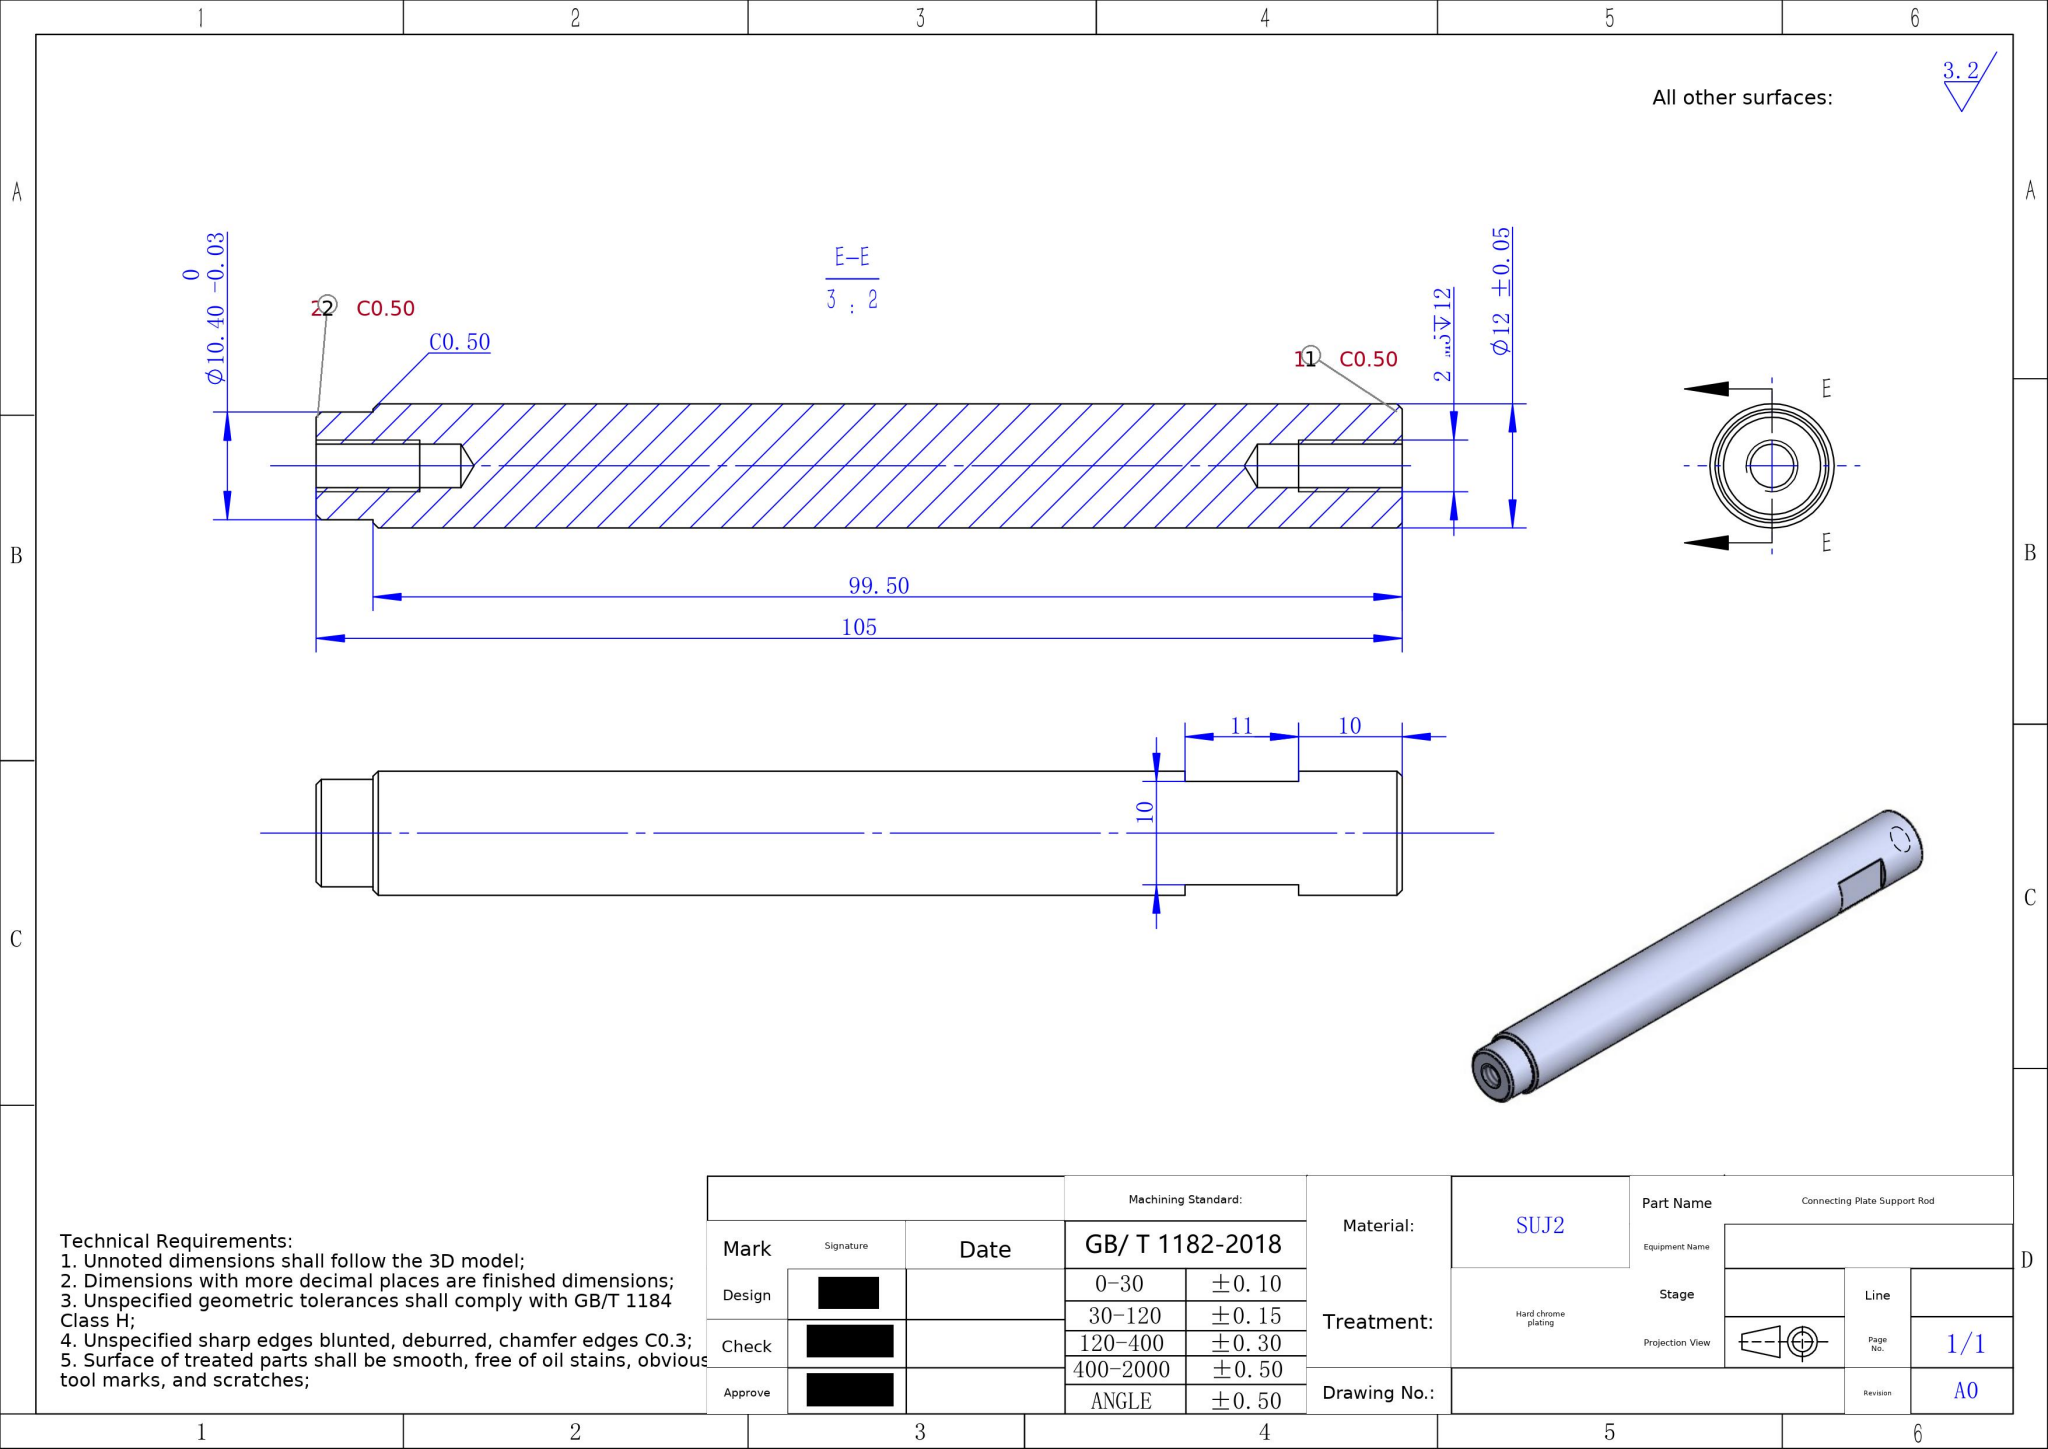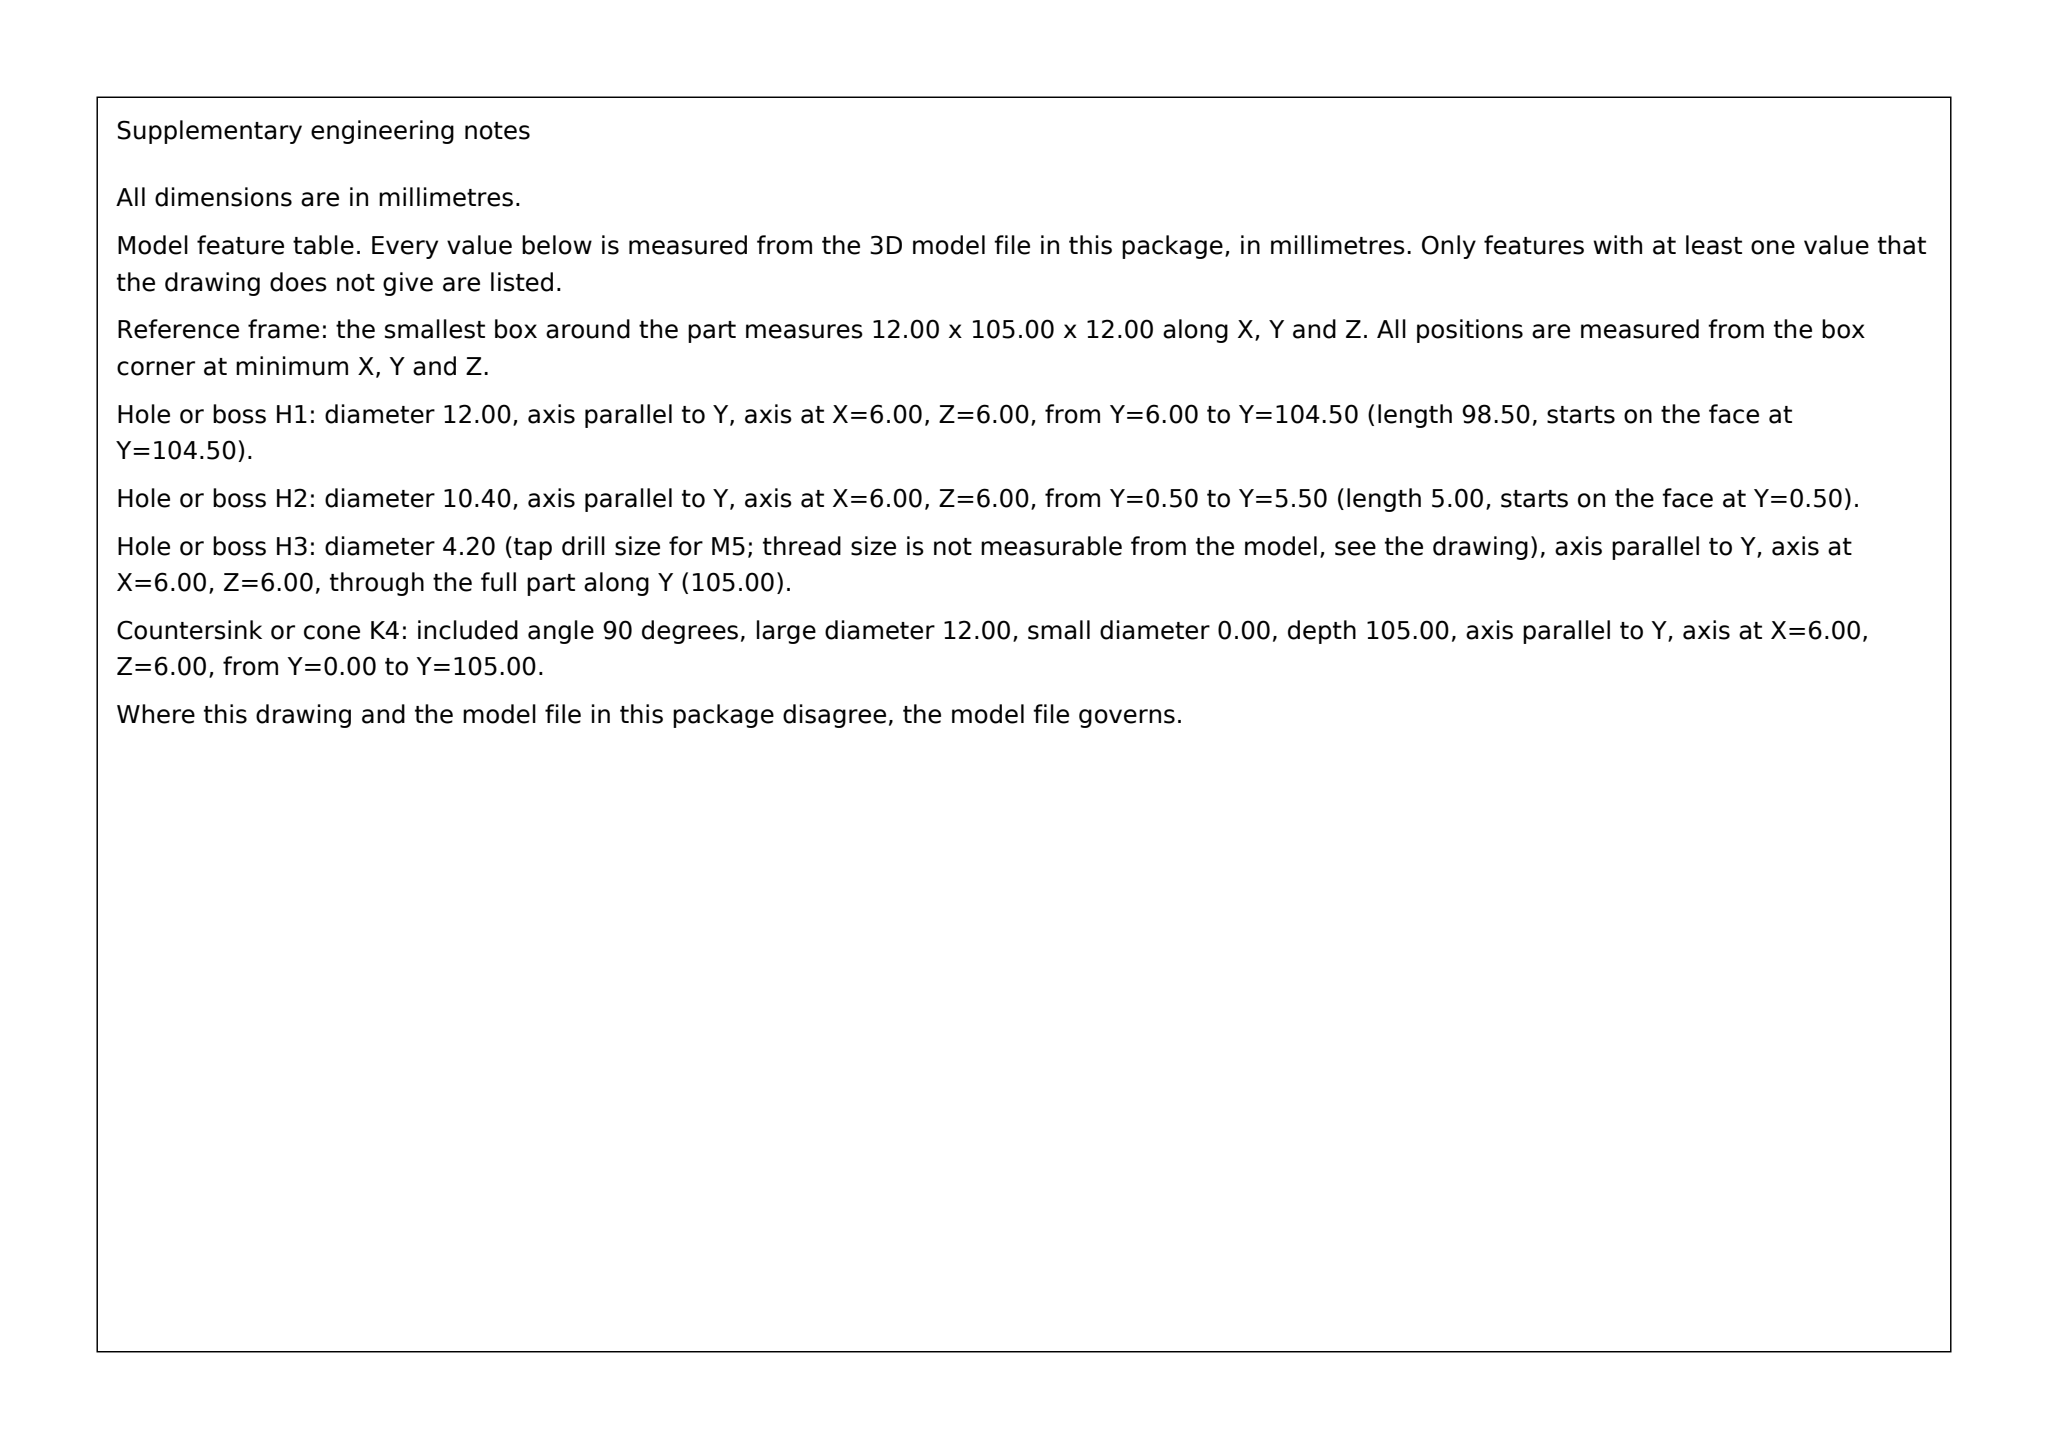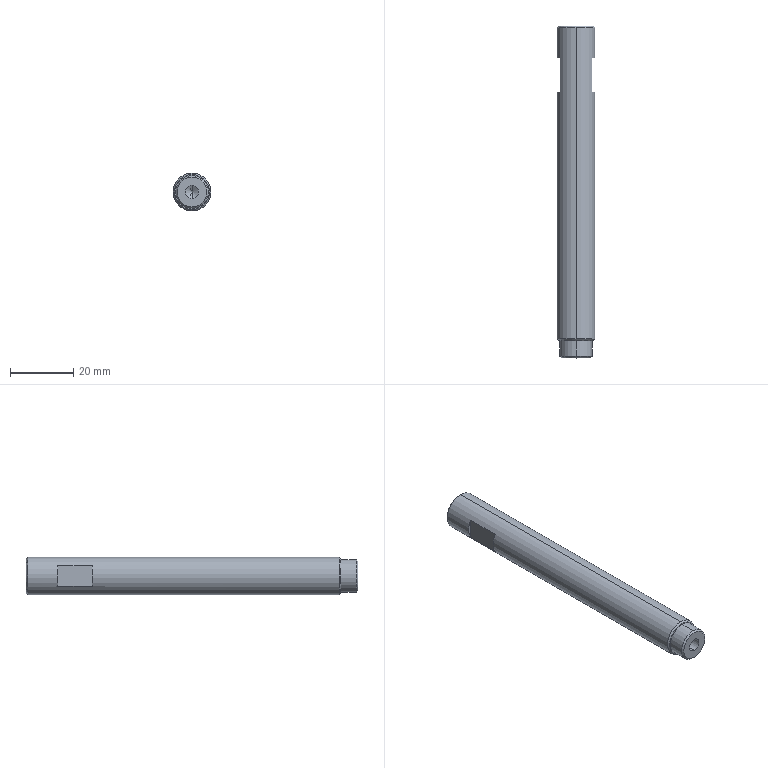Part | SolidWorks | mm | material SUJ2 | 1 solid | 27 faces | box 12 x 105 x 12 mm | volume 11209 mm3 | cone 10 | plane 9 | cylinder 8 | commonest cylinder face diameters 4.2 x4 10.4 x2 12 x2
build123d program:
from build123d import *

# Parameters (mm, degrees)
SKETCH2_W             = 7.253
SKETCH2_H             = 11
CUT_EXTRUDE1_DEPTH    = 15
CHAMFER1_SIZE         = 0.5
M5_TAPPED_HOLE1_D     = 4.2
M5_TAPPED_HOLE1_DEPTH = 14
M5_TAPPED_HOLE1_TIP   = 1.262
M5_TAPPED_HOLE2_D     = 4.2
M5_TAPPED_HOLE2_DEPTH = 14
M5_TAPPED_HOLE2_TIP   = 1.262


with BuildPart() as part:
    # Sketch1 → Revolve1 (revolve)
    with BuildSketch(Plane.XY, mode=Mode.PRIVATE) as revolve1_sk:
        Polygon((0, 0), (6, 0), (6, -10), (6, -21), (6, -99.5), (5.2, -99.5), (5.2, -105), (0, -105), align=None)
    revolve(revolve1_sk.sketch.rotate(Axis((0, 0, 0), (0, 1, 0)), 90), axis=Axis((0, 0, 0), (0, 1, 0)))

    # Sketch2 → Cut-Extrude1 (cut, symmetric)
    with BuildSketch(Plane.XY):
        with Locations((8.626, -15.5)):
            Rectangle(SKETCH2_W, SKETCH2_H)
        with Locations((-8.626, -15.5)):
            Rectangle(SKETCH2_W, SKETCH2_H)
    extrude(amount=CUT_EXTRUDE1_DEPTH, both=True, mode=Mode.SUBTRACT)

    # Chamfer1
    chamfer1_edges = [part.edges().sort_by_distance(p)[0] for p in [
        (0, -105, 5.2),
        (0, -99.5, 6),
        (0, 0, 6),
    ]]
    chamfer(chamfer1_edges, length=CHAMFER1_SIZE)

    # M5 Tapped Hole1
    with Locations(Plane(origin=(0, -105, 0), x_dir=(-1, 0, 0), z_dir=(0, -1, 0))):
        with Locations((0, 0)):
            Hole(M5_TAPPED_HOLE1_D / 2, depth=M5_TAPPED_HOLE1_DEPTH)
            with Locations((0, 0, -(M5_TAPPED_HOLE1_DEPTH + M5_TAPPED_HOLE1_TIP / 2))):  # 118° drill point
                Cone(0, M5_TAPPED_HOLE1_D / 2, M5_TAPPED_HOLE1_TIP, mode=Mode.SUBTRACT)

    # M5 Tapped Hole2
    with Locations(Plane(origin=(0, 0, 0), x_dir=(1, 0, 0), z_dir=(0, 1, 0))):
        with Locations((0, 0)):
            Hole(M5_TAPPED_HOLE2_D / 2, depth=M5_TAPPED_HOLE2_DEPTH)
            with Locations((0, 0, -(M5_TAPPED_HOLE2_DEPTH + M5_TAPPED_HOLE2_TIP / 2))):  # 118° drill point
                Cone(0, M5_TAPPED_HOLE2_D / 2, M5_TAPPED_HOLE2_TIP, mode=Mode.SUBTRACT)


solid = part.part
STEP:
#1=CARTESIAN_POINT('',(0.,-14.,-2.1));
#2=VERTEX_POINT('',#1);
#3=CARTESIAN_POINT('',(0.,-14.,2.1));
#4=VERTEX_POINT('',#3);
#5=CARTESIAN_POINT('',(0.,-14.,0.));
#6=DIRECTION('',(0.,1.,0.));
#7=DIRECTION('',(0.,0.,1.));
#8=AXIS2_PLACEMENT_3D('',#5,#6,#7);
#9=CIRCLE('',#8,2.1);
#10=EDGE_CURVE('',#2,#4,#9,.T.);
#11=ORIENTED_EDGE('',*,*,#10,.F.);
#12=CARTESIAN_POINT('',(0.,0.,-2.1));
#13=VERTEX_POINT('',#12);
#14=CARTESIAN_POINT('',(0.,0.,-2.1));
#15=DIRECTION('',(0.,1.,0.));
#16=VECTOR('',#15,1000.);
#17=LINE('',#14,#16);
#18=EDGE_CURVE('',#2,#13,#17,.T.);
#19=ORIENTED_EDGE('',*,*,#18,.T.);
#20=CARTESIAN_POINT('',(0.,0.,2.1));
#21=VERTEX_POINT('',#20);
#22=CARTESIAN_POINT('',(0.,0.,0.));
#23=DIRECTION('',(0.,1.,0.));
#24=DIRECTION('',(0.,0.,1.));
#25=AXIS2_PLACEMENT_3D('',#22,#23,#24);
#26=CIRCLE('',#25,2.1);
#27=EDGE_CURVE('',#13,#21,#26,.T.);
#28=ORIENTED_EDGE('',*,*,#27,.T.);
#29=CARTESIAN_POINT('',(0.,0.,2.1));
#30=DIRECTION('',(0.,1.,0.));
#31=VECTOR('',#30,1000.);
#32=LINE('',#29,#31);
#33=EDGE_CURVE('',#4,#21,#32,.T.);
#34=ORIENTED_EDGE('',*,*,#33,.F.);
#35=EDGE_LOOP('',(#11,#19,#28,#34));
#36=FACE_OUTER_BOUND('',#35,.T.);
#37=CARTESIAN_POINT('',(0.,0.,0.));
#38=DIRECTION('',(0.,1.,0.));
#39=DIRECTION('',(0.,0.,1.));
#40=AXIS2_PLACEMENT_3D('',#37,#38,#39);
#41=CYLINDRICAL_SURFACE('',#40,2.1);
#42=ADVANCED_FACE('',(#36),#41,.F.);
#43=CARTESIAN_POINT('',(-0.,-15.262,0.));
#44=VERTEX_POINT('',#43);
#45=CARTESIAN_POINT('',(0.,-14.,2.1));
#46=DIRECTION('',(0.,0.515,0.8572));
#47=VECTOR('',#46,1000.);
#48=LINE('',#45,#47);
#49=EDGE_CURVE('',#44,#4,#48,.T.);
#50=ORIENTED_EDGE('',*,*,#49,.F.);
#51=CARTESIAN_POINT('',(0.,-14.,-2.1));
#52=DIRECTION('',(0.,0.515,-0.8572));
#53=VECTOR('',#52,1000.);
#54=LINE('',#51,#53);
#55=EDGE_CURVE('',#44,#2,#54,.T.);
#56=ORIENTED_EDGE('',*,*,#55,.T.);
#57=ORIENTED_EDGE('',*,*,#10,.T.);
#58=EDGE_LOOP('',(#50,#56,#57));
#59=FACE_OUTER_BOUND('',#58,.T.);
#60=CARTESIAN_POINT('',(0.,-14.,0.));
#61=DIRECTION('',(0.,1.,0.));
#62=DIRECTION('',(0.,0.,1.));
#63=AXIS2_PLACEMENT_3D('',#60,#61,#62);
#64=CONICAL_SURFACE('',#63,2.1,1.03);
#65=ADVANCED_FACE('',(#59),#64,.F.);
#66=CARTESIAN_POINT('',(0.,-91.,2.1));
#67=VERTEX_POINT('',#66);
#68=CARTESIAN_POINT('',(0.,-91.,-2.1));
#69=VERTEX_POINT('',#68);
#70=CARTESIAN_POINT('',(0.,-91.,0.));
#71=DIRECTION('',(0.,-1.,0.));
#72=DIRECTION('',(0.,0.,-1.));
#73=AXIS2_PLACEMENT_3D('',#70,#71,#72);
#74=CIRCLE('',#73,2.1);
#75=EDGE_CURVE('',#67,#69,#74,.T.);
#76=ORIENTED_EDGE('',*,*,#75,.F.);
#77=CARTESIAN_POINT('',(0.,-105.,2.1));
#78=VERTEX_POINT('',#77);
#79=CARTESIAN_POINT('',(0.,-105.,2.1));
#80=DIRECTION('',(0.,-1.,0.));
#81=VECTOR('',#80,1000.);
#82=LINE('',#79,#81);
#83=EDGE_CURVE('',#67,#78,#82,.T.);
#84=ORIENTED_EDGE('',*,*,#83,.T.);
#85=CARTESIAN_POINT('',(0.,-105.,-2.1));
#86=VERTEX_POINT('',#85);
#87=CARTESIAN_POINT('',(0.,-105.,0.));
#88=DIRECTION('',(0.,-1.,0.));
#89=DIRECTION('',(0.,0.,-1.));
#90=AXIS2_PLACEMENT_3D('',#87,#88,#89);
#91=CIRCLE('',#90,2.1);
#92=EDGE_CURVE('',#78,#86,#91,.T.);
#93=ORIENTED_EDGE('',*,*,#92,.T.);
#94=CARTESIAN_POINT('',(0.,-105.,-2.1));
#95=DIRECTION('',(0.,-1.,0.));
#96=VECTOR('',#95,1000.);
#97=LINE('',#94,#96);
#98=EDGE_CURVE('',#69,#86,#97,.T.);
#99=ORIENTED_EDGE('',*,*,#98,.F.);
#100=EDGE_LOOP('',(#76,#84,#93,#99));
#101=FACE_OUTER_BOUND('',#100,.T.);
#102=CARTESIAN_POINT('',(0.,-105.,0.));
#103=DIRECTION('',(0.,-1.,0.));
#104=DIRECTION('',(0.,0.,-1.));
#105=AXIS2_PLACEMENT_3D('',#102,#103,#104);
#106=CYLINDRICAL_SURFACE('',#105,2.1);
#107=ADVANCED_FACE('',(#101),#106,.F.);
#108=CARTESIAN_POINT('',(-0.,-89.738,0.));
#109=VERTEX_POINT('',#108);
#110=CARTESIAN_POINT('',(0.,-91.,-2.1));
#111=DIRECTION('',(0.,-0.515,-0.8572));
#112=VECTOR('',#111,1000.);
#113=LINE('',#110,#112);
#114=EDGE_CURVE('',#109,#69,#113,.T.);
#115=ORIENTED_EDGE('',*,*,#114,.F.);
#116=CARTESIAN_POINT('',(0.,-91.,2.1));
#117=DIRECTION('',(0.,-0.515,0.8572));
#118=VECTOR('',#117,1000.);
#119=LINE('',#116,#118);
#120=EDGE_CURVE('',#109,#67,#119,.T.);
#121=ORIENTED_EDGE('',*,*,#120,.T.);
#122=ORIENTED_EDGE('',*,*,#75,.T.);
#123=EDGE_LOOP('',(#115,#121,#122));
#124=FACE_OUTER_BOUND('',#123,.T.);
#125=CARTESIAN_POINT('',(0.,-91.,0.));
#126=DIRECTION('',(0.,-1.,0.));
#127=DIRECTION('',(0.,0.,-1.));
#128=AXIS2_PLACEMENT_3D('',#125,#126,#127);
#129=CONICAL_SURFACE('',#128,2.1,1.03);
#130=ADVANCED_FACE('',(#124),#129,.F.);
#131=CARTESIAN_POINT('',(0.,-0.,5.5));
#132=VERTEX_POINT('',#131);
#133=CARTESIAN_POINT('',(0.,-0.,-5.5));
#134=VERTEX_POINT('',#133);
#135=CARTESIAN_POINT('',(0.,-0.,0.));
#136=DIRECTION('',(0.,1.,0.));
#137=DIRECTION('',(0.,0.,1.));
#138=AXIS2_PLACEMENT_3D('',#135,#136,#137);
#139=CIRCLE('',#138,5.5);
#140=EDGE_CURVE('',#132,#134,#139,.T.);
#141=ORIENTED_EDGE('',*,*,#140,.F.);
#142=CARTESIAN_POINT('',(0.,-0.5,6.));
#143=VERTEX_POINT('',#142);
#144=CARTESIAN_POINT('',(0.,-0.5,6.));
#145=DIRECTION('',(0.,-0.7071,0.7071));
#146=VECTOR('',#145,1000.);
#147=LINE('',#144,#146);
#148=EDGE_CURVE('',#132,#143,#147,.T.);
#149=ORIENTED_EDGE('',*,*,#148,.T.);
#150=CARTESIAN_POINT('',(0.,-0.5,-6.));
#151=VERTEX_POINT('',#150);
#152=CARTESIAN_POINT('',(0.,-0.5,0.));
#153=DIRECTION('',(0.,-1.,0.));
#154=DIRECTION('',(0.,0.,1.));
#155=AXIS2_PLACEMENT_3D('',#152,#153,#154);
#156=CIRCLE('',#155,6.);
#157=EDGE_CURVE('',#151,#143,#156,.T.);
#158=ORIENTED_EDGE('',*,*,#157,.F.);
#159=CARTESIAN_POINT('',(0.,-0.5,-6.));
#160=DIRECTION('',(0.,-0.7071,-0.7071));
#161=VECTOR('',#160,1000.);
#162=LINE('',#159,#161);
#163=EDGE_CURVE('',#134,#151,#162,.T.);
#164=ORIENTED_EDGE('',*,*,#163,.F.);
#165=EDGE_LOOP('',(#141,#149,#158,#164));
#166=FACE_OUTER_BOUND('',#165,.T.);
#167=CARTESIAN_POINT('',(0.,-0.5,0.));
#168=DIRECTION('',(0.,-1.,0.));
#169=DIRECTION('',(0.,0.,-1.));
#170=AXIS2_PLACEMENT_3D('',#167,#168,#169);
#171=CONICAL_SURFACE('',#170,6.,0.7854);
#172=ADVANCED_FACE('',(#166),#171,.T.);
#173=CARTESIAN_POINT('',(0.,-99.5,-5.5));
#174=VERTEX_POINT('',#173);
#175=CARTESIAN_POINT('',(0.,-99.5,5.5));
#176=VERTEX_POINT('',#175);
#177=CARTESIAN_POINT('',(0.,-99.5,0.));
#178=DIRECTION('',(0.,-1.,0.));
#179=DIRECTION('',(0.,0.,-1.));
#180=AXIS2_PLACEMENT_3D('',#177,#178,#179);
#181=CIRCLE('',#180,5.5);
#182=EDGE_CURVE('',#174,#176,#181,.T.);
#183=ORIENTED_EDGE('',*,*,#182,.F.);
#184=CARTESIAN_POINT('',(0.,-99.,-6.));
#185=VERTEX_POINT('',#184);
#186=CARTESIAN_POINT('',(0.,-99.5,-5.5));
#187=DIRECTION('',(0.,0.7071,-0.7071));
#188=VECTOR('',#187,1000.);
#189=LINE('',#186,#188);
#190=EDGE_CURVE('',#174,#185,#189,.T.);
#191=ORIENTED_EDGE('',*,*,#190,.T.);
#192=CARTESIAN_POINT('',(0.,-99.,6.));
#193=VERTEX_POINT('',#192);
#194=CARTESIAN_POINT('',(0.,-99.,0.));
#195=DIRECTION('',(0.,1.,0.));
#196=DIRECTION('',(0.,0.,-1.));
#197=AXIS2_PLACEMENT_3D('',#194,#195,#196);
#198=CIRCLE('',#197,6.);
#199=EDGE_CURVE('',#193,#185,#198,.T.);
#200=ORIENTED_EDGE('',*,*,#199,.F.);
#201=CARTESIAN_POINT('',(0.,-99.5,5.5));
#202=DIRECTION('',(0.,0.7071,0.7071));
#203=VECTOR('',#202,1000.);
#204=LINE('',#201,#203);
#205=EDGE_CURVE('',#176,#193,#204,.T.);
#206=ORIENTED_EDGE('',*,*,#205,.F.);
#207=EDGE_LOOP('',(#183,#191,#200,#206));
#208=FACE_OUTER_BOUND('',#207,.T.);
#209=CARTESIAN_POINT('',(0.,-99.5,0.));
#210=DIRECTION('',(0.,1.,0.));
#211=DIRECTION('',(0.,0.,1.));
#212=AXIS2_PLACEMENT_3D('',#209,#210,#211);
#213=CONICAL_SURFACE('',#212,5.5,0.7854);
#214=ADVANCED_FACE('',(#208),#213,.T.);
#215=CARTESIAN_POINT('',(0.,-105.,-4.7));
#216=VERTEX_POINT('',#215);
#217=CARTESIAN_POINT('',(0.,-105.,4.7));
#218=VERTEX_POINT('',#217);
#219=CARTESIAN_POINT('',(0.,-105.,0.));
#220=DIRECTION('',(0.,-1.,0.));
#221=DIRECTION('',(0.,0.,-1.));
#222=AXIS2_PLACEMENT_3D('',#219,#220,#221);
#223=CIRCLE('',#222,4.7);
#224=EDGE_CURVE('',#216,#218,#223,.T.);
#225=ORIENTED_EDGE('',*,*,#224,.F.);
#226=CARTESIAN_POINT('',(0.,-104.5,-5.2));
#227=VERTEX_POINT('',#226);
#228=CARTESIAN_POINT('',(0.,-105.,-4.7));
#229=DIRECTION('',(0.,0.7071,-0.7071));
#230=VECTOR('',#229,1000.);
#231=LINE('',#228,#230);
#232=EDGE_CURVE('',#216,#227,#231,.T.);
#233=ORIENTED_EDGE('',*,*,#232,.T.);
#234=CARTESIAN_POINT('',(0.,-104.5,5.2));
#235=VERTEX_POINT('',#234);
#236=CARTESIAN_POINT('',(0.,-104.5,0.));
#237=DIRECTION('',(0.,1.,0.));
#238=DIRECTION('',(0.,0.,-1.));
#239=AXIS2_PLACEMENT_3D('',#236,#237,#238);
#240=CIRCLE('',#239,5.2);
#241=EDGE_CURVE('',#235,#227,#240,.T.);
#242=ORIENTED_EDGE('',*,*,#241,.F.);
#243=CARTESIAN_POINT('',(0.,-105.,4.7));
#244=DIRECTION('',(0.,0.7071,0.7071));
#245=VECTOR('',#244,1000.);
#246=LINE('',#243,#245);
#247=EDGE_CURVE('',#218,#235,#246,.T.);
#248=ORIENTED_EDGE('',*,*,#247,.F.);
#249=EDGE_LOOP('',(#225,#233,#242,#248));
#250=FACE_OUTER_BOUND('',#249,.T.);
#251=CARTESIAN_POINT('',(0.,-105.,0.));
#252=DIRECTION('',(0.,1.,0.));
#253=DIRECTION('',(0.,0.,1.));
#254=AXIS2_PLACEMENT_3D('',#251,#252,#253);
#255=CONICAL_SURFACE('',#254,4.7,0.7854);
#256=ADVANCED_FACE('',(#250),#255,.T.);
#257=CARTESIAN_POINT('',(0.,-99.5,-5.2));
#258=VERTEX_POINT('',#257);
#259=CARTESIAN_POINT('',(0.,-99.5,5.2));
#260=VERTEX_POINT('',#259);
#261=CARTESIAN_POINT('',(0.,-99.5,0.));
#262=DIRECTION('',(0.,-1.,0.));
#263=DIRECTION('',(0.,0.,-1.));
#264=AXIS2_PLACEMENT_3D('',#261,#262,#263);
#265=CIRCLE('',#264,5.2);
#266=EDGE_CURVE('',#258,#260,#265,.T.);
#267=ORIENTED_EDGE('',*,*,#266,.T.);
#268=CARTESIAN_POINT('',(0.,0.,5.2));
#269=DIRECTION('',(0.,-1.,0.));
#270=VECTOR('',#269,1000.);
#271=LINE('',#268,#270);
#272=EDGE_CURVE('',#260,#235,#271,.T.);
#273=ORIENTED_EDGE('',*,*,#272,.T.);
#274=ORIENTED_EDGE('',*,*,#241,.T.);
#275=CARTESIAN_POINT('',(0.,0.,-5.2));
#276=DIRECTION('',(0.,-1.,0.));
#277=VECTOR('',#276,1000.);
#278=LINE('',#275,#277);
#279=EDGE_CURVE('',#258,#227,#278,.T.);
#280=ORIENTED_EDGE('',*,*,#279,.F.);
#281=EDGE_LOOP('',(#267,#273,#274,#280));
#282=FACE_OUTER_BOUND('',#281,.T.);
#283=CARTESIAN_POINT('',(0.,0.,0.));
#284=DIRECTION('',(0.,-1.,0.));
#285=DIRECTION('',(0.,0.,-1.));
#286=AXIS2_PLACEMENT_3D('',#283,#284,#285);
#287=CYLINDRICAL_SURFACE('',#286,5.2);
#288=ADVANCED_FACE('',(#282),#287,.T.);
#289=CARTESIAN_POINT('',(5.,-21.,3.317));
#290=VERTEX_POINT('',#289);
#291=CARTESIAN_POINT('',(5.,-21.,-3.317));
#292=VERTEX_POINT('',#291);
#293=CARTESIAN_POINT('',(0.,-21.,0.));
#294=DIRECTION('',(0.,1.,0.));
#295=DIRECTION('',(-0.,0.,-1.));
#296=AXIS2_PLACEMENT_3D('',#293,#294,#295);
#297=CIRCLE('',#296,6.);
#298=EDGE_CURVE('',#290,#292,#297,.T.);
#299=ORIENTED_EDGE('',*,*,#298,.F.);
#300=CARTESIAN_POINT('',(5.,-10.,3.317));
#301=VERTEX_POINT('',#300);
#302=CARTESIAN_POINT('',(5.,0.,3.317));
#303=DIRECTION('',(0.,-1.,0.));
#304=VECTOR('',#303,1000.);
#305=LINE('',#302,#304);
#306=EDGE_CURVE('',#301,#290,#305,.T.);
#307=ORIENTED_EDGE('',*,*,#306,.F.);
#308=CARTESIAN_POINT('',(5.,-10.,-3.317));
#309=VERTEX_POINT('',#308);
#310=CARTESIAN_POINT('',(0.,-10.,0.));
#311=DIRECTION('',(-0.,-1.,0.));
#312=DIRECTION('',(-1.,0.,0.));
#313=AXIS2_PLACEMENT_3D('',#310,#311,#312);
#314=CIRCLE('',#313,6.);
#315=EDGE_CURVE('',#309,#301,#314,.T.);
#316=ORIENTED_EDGE('',*,*,#315,.F.);
#317=CARTESIAN_POINT('',(5.,0.,-3.317));
#318=DIRECTION('',(0.,1.,0.));
#319=VECTOR('',#318,1000.);
#320=LINE('',#317,#319);
#321=EDGE_CURVE('',#292,#309,#320,.T.);
#322=ORIENTED_EDGE('',*,*,#321,.F.);
#323=EDGE_LOOP('',(#299,#307,#316,#322));
#324=FACE_BOUND('',#323,.T.);
#325=ORIENTED_EDGE('',*,*,#157,.T.);
#326=CARTESIAN_POINT('',(0.,0.,6.));
#327=DIRECTION('',(0.,-1.,0.));
#328=VECTOR('',#327,1000.);
#329=LINE('',#326,#328);
#330=EDGE_CURVE('',#143,#193,#329,.T.);
#331=ORIENTED_EDGE('',*,*,#330,.T.);
#332=ORIENTED_EDGE('',*,*,#199,.T.);
#333=CARTESIAN_POINT('',(0.,0.,-6.));
#334=DIRECTION('',(0.,-1.,0.));
#335=VECTOR('',#334,1000.);
#336=LINE('',#333,#335);
#337=EDGE_CURVE('',#151,#185,#336,.T.);
#338=ORIENTED_EDGE('',*,*,#337,.F.);
#339=EDGE_LOOP('',(#325,#331,#332,#338));
#340=FACE_OUTER_BOUND('',#339,.T.);
#341=CARTESIAN_POINT('',(0.,0.,0.));
#342=DIRECTION('',(0.,-1.,0.));
#343=DIRECTION('',(0.,0.,-1.));
#344=AXIS2_PLACEMENT_3D('',#341,#342,#343);
#345=CYLINDRICAL_SURFACE('',#344,6.);
#346=ADVANCED_FACE('',(#324,#340),#345,.T.);
#347=CARTESIAN_POINT('',(0.,0.,0.));
#348=DIRECTION('',(0.,1.,0.));
#349=DIRECTION('',(0.,0.,1.));
#350=AXIS2_PLACEMENT_3D('',#347,#348,#349);
#351=CIRCLE('',#350,2.1);
#352=EDGE_CURVE('',#21,#13,#351,.T.);
#353=ORIENTED_EDGE('',*,*,#352,.F.);
#354=ORIENTED_EDGE('',*,*,#27,.F.);
#355=EDGE_LOOP('',(#353,#354));
#356=FACE_BOUND('',#355,.T.);
#357=CARTESIAN_POINT('',(0.,-0.,0.));
#358=DIRECTION('',(0.,1.,0.));
#359=DIRECTION('',(0.,0.,1.));
#360=AXIS2_PLACEMENT_3D('',#357,#358,#359);
#361=CIRCLE('',#360,5.5);
#362=EDGE_CURVE('',#134,#132,#361,.T.);
#363=ORIENTED_EDGE('',*,*,#362,.T.);
#364=ORIENTED_EDGE('',*,*,#140,.T.);
#365=EDGE_LOOP('',(#363,#364));
#366=FACE_OUTER_BOUND('',#365,.T.);
#367=CARTESIAN_POINT('',(0.,-0.,0.));
#368=DIRECTION('',(0.,1.,0.));
#369=DIRECTION('',(0.,0.,1.));
#370=AXIS2_PLACEMENT_3D('',#367,#368,#369);
#371=PLANE('',#370);
#372=ADVANCED_FACE('',(#356,#366),#371,.T.);
#373=ORIENTED_EDGE('',*,*,#330,.F.);
#374=CARTESIAN_POINT('',(0.,-0.5,0.));
#375=DIRECTION('',(0.,-1.,0.));
#376=DIRECTION('',(0.,0.,1.));
#377=AXIS2_PLACEMENT_3D('',#374,#375,#376);
#378=CIRCLE('',#377,6.);
#379=EDGE_CURVE('',#143,#151,#378,.T.);
#380=ORIENTED_EDGE('',*,*,#379,.T.);
#381=ORIENTED_EDGE('',*,*,#337,.T.);
#382=CARTESIAN_POINT('',(0.,-99.,0.));
#383=DIRECTION('',(0.,1.,0.));
#384=DIRECTION('',(0.,0.,-1.));
#385=AXIS2_PLACEMENT_3D('',#382,#383,#384);
#386=CIRCLE('',#385,6.);
#387=EDGE_CURVE('',#185,#193,#386,.T.);
#388=ORIENTED_EDGE('',*,*,#387,.T.);
#389=EDGE_LOOP('',(#373,#380,#381,#388));
#390=FACE_OUTER_BOUND('',#389,.T.);
#391=CARTESIAN_POINT('',(-5.,-10.,3.317));
#392=VERTEX_POINT('',#391);
#393=CARTESIAN_POINT('',(-5.,-10.,-3.317));
#394=VERTEX_POINT('',#393);
#395=CARTESIAN_POINT('',(0.,-10.,0.));
#396=DIRECTION('',(0.,-1.,0.));
#397=DIRECTION('',(-1.,-0.,0.));
#398=AXIS2_PLACEMENT_3D('',#395,#396,#397);
#399=CIRCLE('',#398,6.);
#400=EDGE_CURVE('',#392,#394,#399,.T.);
#401=ORIENTED_EDGE('',*,*,#400,.F.);
#402=CARTESIAN_POINT('',(-5.,-21.,3.317));
#403=VERTEX_POINT('',#402);
#404=CARTESIAN_POINT('',(-5.,0.,3.317));
#405=DIRECTION('',(0.,1.,0.));
#406=VECTOR('',#405,1000.);
#407=LINE('',#404,#406);
#408=EDGE_CURVE('',#403,#392,#407,.T.);
#409=ORIENTED_EDGE('',*,*,#408,.F.);
#410=CARTESIAN_POINT('',(-5.,-21.,-3.317));
#411=VERTEX_POINT('',#410);
#412=CARTESIAN_POINT('',(0.,-21.,0.));
#413=DIRECTION('',(0.,1.,0.));
#414=DIRECTION('',(0.,0.,-1.));
#415=AXIS2_PLACEMENT_3D('',#412,#413,#414);
#416=CIRCLE('',#415,6.);
#417=EDGE_CURVE('',#411,#403,#416,.T.);
#418=ORIENTED_EDGE('',*,*,#417,.F.);
#419=CARTESIAN_POINT('',(-5.,0.,-3.317));
#420=DIRECTION('',(0.,-1.,0.));
#421=VECTOR('',#420,1000.);
#422=LINE('',#419,#421);
#423=EDGE_CURVE('',#394,#411,#422,.T.);
#424=ORIENTED_EDGE('',*,*,#423,.F.);
#425=EDGE_LOOP('',(#401,#409,#418,#424));
#426=FACE_BOUND('',#425,.T.);
#427=CARTESIAN_POINT('',(0.,0.,0.));
#428=DIRECTION('',(0.,-1.,0.));
#429=DIRECTION('',(0.,0.,-1.));
#430=AXIS2_PLACEMENT_3D('',#427,#428,#429);
#431=CYLINDRICAL_SURFACE('',#430,6.);
#432=ADVANCED_FACE('',(#390,#426),#431,.T.);
#433=CARTESIAN_POINT('',(0.,-99.5,0.));
#434=DIRECTION('',(0.,-1.,0.));
#435=DIRECTION('',(0.,0.,-1.));
#436=AXIS2_PLACEMENT_3D('',#433,#434,#435);
#437=CIRCLE('',#436,5.5);
#438=EDGE_CURVE('',#176,#174,#437,.T.);
#439=ORIENTED_EDGE('',*,*,#438,.T.);
#440=ORIENTED_EDGE('',*,*,#182,.T.);
#441=EDGE_LOOP('',(#439,#440));
#442=FACE_OUTER_BOUND('',#441,.T.);
#443=ORIENTED_EDGE('',*,*,#266,.F.);
#444=CARTESIAN_POINT('',(0.,-99.5,0.));
#445=DIRECTION('',(0.,-1.,0.));
#446=DIRECTION('',(0.,0.,-1.));
#447=AXIS2_PLACEMENT_3D('',#444,#445,#446);
#448=CIRCLE('',#447,5.2);
#449=EDGE_CURVE('',#260,#258,#448,.T.);
#450=ORIENTED_EDGE('',*,*,#449,.F.);
#451=EDGE_LOOP('',(#443,#450));
#452=FACE_BOUND('',#451,.T.);
#453=CARTESIAN_POINT('',(6.,-99.5,0.));
#454=DIRECTION('',(0.,-1.,0.));
#455=DIRECTION('',(0.,0.,-1.));
#456=AXIS2_PLACEMENT_3D('',#453,#454,#455);
#457=PLANE('',#456);
#458=ADVANCED_FACE('',(#442,#452),#457,.T.);
#459=ORIENTED_EDGE('',*,*,#272,.F.);
#460=ORIENTED_EDGE('',*,*,#449,.T.);
#461=ORIENTED_EDGE('',*,*,#279,.T.);
#462=CARTESIAN_POINT('',(0.,-104.5,0.));
#463=DIRECTION('',(0.,1.,0.));
#464=DIRECTION('',(0.,0.,-1.));
#465=AXIS2_PLACEMENT_3D('',#462,#463,#464);
#466=CIRCLE('',#465,5.2);
#467=EDGE_CURVE('',#227,#235,#466,.T.);
#468=ORIENTED_EDGE('',*,*,#467,.T.);
#469=EDGE_LOOP('',(#459,#460,#461,#468));
#470=FACE_OUTER_BOUND('',#469,.T.);
#471=CARTESIAN_POINT('',(0.,0.,0.));
#472=DIRECTION('',(0.,-1.,0.));
#473=DIRECTION('',(0.,0.,-1.));
#474=AXIS2_PLACEMENT_3D('',#471,#472,#473);
#475=CYLINDRICAL_SURFACE('',#474,5.2);
#476=ADVANCED_FACE('',(#470),#475,.T.);
#477=CARTESIAN_POINT('',(0.,-105.,0.));
#478=DIRECTION('',(0.,-1.,0.));
#479=DIRECTION('',(0.,0.,-1.));
#480=AXIS2_PLACEMENT_3D('',#477,#478,#479);
#481=CIRCLE('',#480,2.1);
#482=EDGE_CURVE('',#86,#78,#481,.T.);
#483=ORIENTED_EDGE('',*,*,#482,.F.);
#484=ORIENTED_EDGE('',*,*,#92,.F.);
#485=EDGE_LOOP('',(#483,#484));
#486=FACE_BOUND('',#485,.T.);
#487=CARTESIAN_POINT('',(0.,-105.,0.));
#488=DIRECTION('',(0.,-1.,0.));
#489=DIRECTION('',(0.,0.,-1.));
#490=AXIS2_PLACEMENT_3D('',#487,#488,#489);
#491=CIRCLE('',#490,4.7);
#492=EDGE_CURVE('',#218,#216,#491,.T.);
#493=ORIENTED_EDGE('',*,*,#492,.T.);
#494=ORIENTED_EDGE('',*,*,#224,.T.);
#495=EDGE_LOOP('',(#493,#494));
#496=FACE_OUTER_BOUND('',#495,.T.);
#497=CARTESIAN_POINT('',(5.2,-105.,0.));
#498=DIRECTION('',(0.,-1.,0.));
#499=DIRECTION('',(0.,0.,-1.));
#500=AXIS2_PLACEMENT_3D('',#497,#498,#499);
#501=PLANE('',#500);
#502=ADVANCED_FACE('',(#486,#496),#501,.T.);
#503=ORIENTED_EDGE('',*,*,#400,.T.);
#504=CARTESIAN_POINT('',(-5.,-10.,-15.));
#505=DIRECTION('',(0.,0.,1.));
#506=VECTOR('',#505,1000.);
#507=LINE('',#504,#506);
#508=EDGE_CURVE('',#394,#392,#507,.T.);
#509=ORIENTED_EDGE('',*,*,#508,.T.);
#510=EDGE_LOOP('',(#503,#509));
#511=FACE_OUTER_BOUND('',#510,.T.);
#512=CARTESIAN_POINT('',(-12.253,-10.,-15.));
#513=DIRECTION('',(-0.,1.,0.));
#514=DIRECTION('',(-1.,-0.,0.));
#515=AXIS2_PLACEMENT_3D('',#512,#513,#514);
#516=PLANE('',#515);
#517=ADVANCED_FACE('',(#511),#516,.F.);
#518=ORIENTED_EDGE('',*,*,#408,.T.);
#519=ORIENTED_EDGE('',*,*,#508,.F.);
#520=ORIENTED_EDGE('',*,*,#423,.T.);
#521=CARTESIAN_POINT('',(-5.,-21.,-15.));
#522=DIRECTION('',(0.,0.,1.));
#523=VECTOR('',#522,1000.);
#524=LINE('',#521,#523);
#525=EDGE_CURVE('',#411,#403,#524,.T.);
#526=ORIENTED_EDGE('',*,*,#525,.T.);
#527=EDGE_LOOP('',(#518,#519,#520,#526));
#528=FACE_OUTER_BOUND('',#527,.T.);
#529=CARTESIAN_POINT('',(-5.,-10.,-15.));
#530=DIRECTION('',(1.,-0.,0.));
#531=DIRECTION('',(0.,1.,0.));
#532=AXIS2_PLACEMENT_3D('',#529,#530,#531);
#533=PLANE('',#532);
#534=ADVANCED_FACE('',(#528),#533,.F.);
#535=ORIENTED_EDGE('',*,*,#417,.T.);
#536=ORIENTED_EDGE('',*,*,#525,.F.);
#537=EDGE_LOOP('',(#535,#536));
#538=FACE_OUTER_BOUND('',#537,.T.);
#539=CARTESIAN_POINT('',(-12.253,-21.,-15.));
#540=DIRECTION('',(0.,-1.,0.));
#541=DIRECTION('',(0.,0.,-1.));
#542=AXIS2_PLACEMENT_3D('',#539,#540,#541);
#543=PLANE('',#542);
#544=ADVANCED_FACE('',(#538),#543,.F.);
#545=ORIENTED_EDGE('',*,*,#298,.T.);
#546=CARTESIAN_POINT('',(5.,-21.,-15.));
#547=DIRECTION('',(0.,0.,1.));
#548=VECTOR('',#547,1000.);
#549=LINE('',#546,#548);
#550=EDGE_CURVE('',#292,#290,#549,.T.);
#551=ORIENTED_EDGE('',*,*,#550,.T.);
#552=EDGE_LOOP('',(#545,#551));
#553=FACE_OUTER_BOUND('',#552,.T.);
#554=CARTESIAN_POINT('',(12.253,-21.,-15.));
#555=DIRECTION('',(0.,-1.,0.));
#556=DIRECTION('',(0.,0.,-1.));
#557=AXIS2_PLACEMENT_3D('',#554,#555,#556);
#558=PLANE('',#557);
#559=ADVANCED_FACE('',(#553),#558,.F.);
#560=ORIENTED_EDGE('',*,*,#321,.T.);
#561=CARTESIAN_POINT('',(5.,-10.,-15.));
#562=DIRECTION('',(0.,0.,1.));
#563=VECTOR('',#562,1000.);
#564=LINE('',#561,#563);
#565=EDGE_CURVE('',#309,#301,#564,.T.);
#566=ORIENTED_EDGE('',*,*,#565,.T.);
#567=ORIENTED_EDGE('',*,*,#306,.T.);
#568=ORIENTED_EDGE('',*,*,#550,.F.);
#569=EDGE_LOOP('',(#560,#566,#567,#568));
#570=FACE_OUTER_BOUND('',#569,.T.);
#571=CARTESIAN_POINT('',(5.,-10.,-15.));
#572=DIRECTION('',(-1.,-0.,0.));
#573=DIRECTION('',(0.,-1.,0.));
#574=AXIS2_PLACEMENT_3D('',#571,#572,#573);
#575=PLANE('',#574);
#576=ADVANCED_FACE('',(#570),#575,.F.);
#577=ORIENTED_EDGE('',*,*,#315,.T.);
#578=ORIENTED_EDGE('',*,*,#565,.F.);
#579=EDGE_LOOP('',(#577,#578));
#580=FACE_OUTER_BOUND('',#579,.T.);
#581=CARTESIAN_POINT('',(12.253,-10.,-15.));
#582=DIRECTION('',(0.,1.,0.));
#583=DIRECTION('',(-1.,0.,0.));
#584=AXIS2_PLACEMENT_3D('',#581,#582,#583);
#585=PLANE('',#584);
#586=ADVANCED_FACE('',(#580),#585,.F.);
#587=ORIENTED_EDGE('',*,*,#232,.F.);
#588=ORIENTED_EDGE('',*,*,#492,.F.);
#589=ORIENTED_EDGE('',*,*,#247,.T.);
#590=ORIENTED_EDGE('',*,*,#467,.F.);
#591=EDGE_LOOP('',(#587,#588,#589,#590));
#592=FACE_OUTER_BOUND('',#591,.T.);
#593=CARTESIAN_POINT('',(0.,-105.,0.));
#594=DIRECTION('',(0.,1.,0.));
#595=DIRECTION('',(0.,0.,1.));
#596=AXIS2_PLACEMENT_3D('',#593,#594,#595);
#597=CONICAL_SURFACE('',#596,4.7,0.7854);
#598=ADVANCED_FACE('',(#592),#597,.T.);
#599=ORIENTED_EDGE('',*,*,#190,.F.);
#600=ORIENTED_EDGE('',*,*,#438,.F.);
#601=ORIENTED_EDGE('',*,*,#205,.T.);
#602=ORIENTED_EDGE('',*,*,#387,.F.);
#603=EDGE_LOOP('',(#599,#600,#601,#602));
#604=FACE_OUTER_BOUND('',#603,.T.);
#605=CARTESIAN_POINT('',(0.,-99.5,0.));
#606=DIRECTION('',(0.,1.,0.));
#607=DIRECTION('',(0.,0.,1.));
#608=AXIS2_PLACEMENT_3D('',#605,#606,#607);
#609=CONICAL_SURFACE('',#608,5.5,0.7854);
#610=ADVANCED_FACE('',(#604),#609,.T.);
#611=ORIENTED_EDGE('',*,*,#148,.F.);
#612=ORIENTED_EDGE('',*,*,#362,.F.);
#613=ORIENTED_EDGE('',*,*,#163,.T.);
#614=ORIENTED_EDGE('',*,*,#379,.F.);
#615=EDGE_LOOP('',(#611,#612,#613,#614));
#616=FACE_OUTER_BOUND('',#615,.T.);
#617=CARTESIAN_POINT('',(0.,-0.5,0.));
#618=DIRECTION('',(0.,-1.,0.));
#619=DIRECTION('',(0.,0.,-1.));
#620=AXIS2_PLACEMENT_3D('',#617,#618,#619);
#621=CONICAL_SURFACE('',#620,6.,0.7854);
#622=ADVANCED_FACE('',(#616),#621,.T.);
#623=ORIENTED_EDGE('',*,*,#120,.F.);
#624=ORIENTED_EDGE('',*,*,#114,.T.);
#625=CARTESIAN_POINT('',(0.,-91.,0.));
#626=DIRECTION('',(0.,-1.,0.));
#627=DIRECTION('',(0.,0.,-1.));
#628=AXIS2_PLACEMENT_3D('',#625,#626,#627);
#629=CIRCLE('',#628,2.1);
#630=EDGE_CURVE('',#69,#67,#629,.T.);
#631=ORIENTED_EDGE('',*,*,#630,.T.);
#632=EDGE_LOOP('',(#623,#624,#631));
#633=FACE_OUTER_BOUND('',#632,.T.);
#634=CARTESIAN_POINT('',(0.,-91.,0.));
#635=DIRECTION('',(0.,-1.,0.));
#636=DIRECTION('',(0.,0.,-1.));
#637=AXIS2_PLACEMENT_3D('',#634,#635,#636);
#638=CONICAL_SURFACE('',#637,2.1,1.03);
#639=ADVANCED_FACE('',(#633),#638,.F.);
#640=ORIENTED_EDGE('',*,*,#83,.F.);
#641=ORIENTED_EDGE('',*,*,#630,.F.);
#642=ORIENTED_EDGE('',*,*,#98,.T.);
#643=ORIENTED_EDGE('',*,*,#482,.T.);
#644=EDGE_LOOP('',(#640,#641,#642,#643));
#645=FACE_OUTER_BOUND('',#644,.T.);
#646=CARTESIAN_POINT('',(0.,-105.,0.));
#647=DIRECTION('',(0.,-1.,0.));
#648=DIRECTION('',(0.,0.,-1.));
#649=AXIS2_PLACEMENT_3D('',#646,#647,#648);
#650=CYLINDRICAL_SURFACE('',#649,2.1);
#651=ADVANCED_FACE('',(#645),#650,.F.);
#652=ORIENTED_EDGE('',*,*,#55,.F.);
#653=ORIENTED_EDGE('',*,*,#49,.T.);
#654=CARTESIAN_POINT('',(0.,-14.,0.));
#655=DIRECTION('',(0.,1.,0.));
#656=DIRECTION('',(0.,0.,1.));
#657=AXIS2_PLACEMENT_3D('',#654,#655,#656);
#658=CIRCLE('',#657,2.1);
#659=EDGE_CURVE('',#4,#2,#658,.T.);
#660=ORIENTED_EDGE('',*,*,#659,.T.);
#661=EDGE_LOOP('',(#652,#653,#660));
#662=FACE_OUTER_BOUND('',#661,.T.);
#663=CARTESIAN_POINT('',(0.,-14.,0.));
#664=DIRECTION('',(0.,1.,0.));
#665=DIRECTION('',(0.,0.,1.));
#666=AXIS2_PLACEMENT_3D('',#663,#664,#665);
#667=CONICAL_SURFACE('',#666,2.1,1.03);
#668=ADVANCED_FACE('',(#662),#667,.F.);
#669=ORIENTED_EDGE('',*,*,#18,.F.);
#670=ORIENTED_EDGE('',*,*,#659,.F.);
#671=ORIENTED_EDGE('',*,*,#33,.T.);
#672=ORIENTED_EDGE('',*,*,#352,.T.);
#673=EDGE_LOOP('',(#669,#670,#671,#672));
#674=FACE_OUTER_BOUND('',#673,.T.);
#675=CARTESIAN_POINT('',(0.,0.,0.));
#676=DIRECTION('',(0.,1.,0.));
#677=DIRECTION('',(0.,0.,1.));
#678=AXIS2_PLACEMENT_3D('',#675,#676,#677);
#679=CYLINDRICAL_SURFACE('',#678,2.1);
#680=ADVANCED_FACE('',(#674),#679,.F.);
#681=CLOSED_SHELL('',(#42,#65,#107,#130,#172,#214,#256,#288,#346,#372,#432,#458,#476,#502,#517,#534,#544,#559,#576,#586,#598,#610,#622,#639,#651,#668,#680));
#682=MANIFOLD_SOLID_BREP('',#681);
#683=CARTESIAN_POINT('',(0.,0.,0.));
#684=DIRECTION('',(0.,0.,1.));
#685=DIRECTION('',(1.,0.,0.));
#686=AXIS2_PLACEMENT_3D('',#683,#684,#685);
#687=(LENGTH_UNIT()NAMED_UNIT(*)SI_UNIT(.MILLI.,.METRE.));
#688=UNCERTAINTY_MEASURE_WITH_UNIT(LENGTH_MEASURE(0.00001),#687,'','');
#689=(NAMED_UNIT(*)PLANE_ANGLE_UNIT()SI_UNIT($,.RADIAN.));
#690=(NAMED_UNIT(*)SI_UNIT($,.STERADIAN.)SOLID_ANGLE_UNIT());
#691=(GEOMETRIC_REPRESENTATION_CONTEXT(3)GLOBAL_UNCERTAINTY_ASSIGNED_CONTEXT((#688))GLOBAL_UNIT_ASSIGNED_CONTEXT((#687,#689,#690))REPRESENTATION_CONTEXT('',''));
#692=ADVANCED_BREP_SHAPE_REPRESENTATION('',(#682,#686),#691);